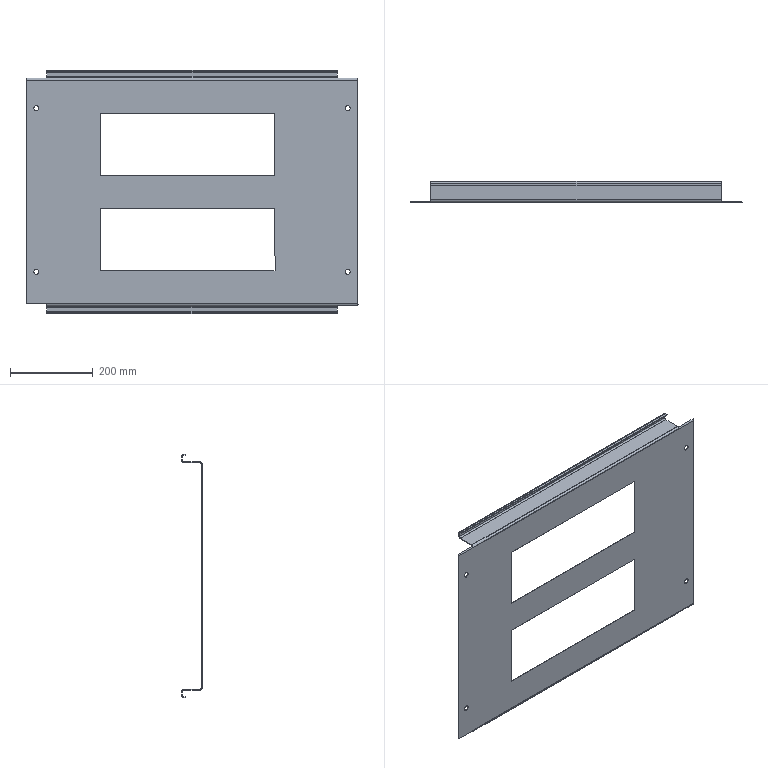Component | SolidWorks | LowerBaffle-2 | 1 solid | 71 faces | volume 816647 mm3 | plane 51 | cylinder 20 | commonest cylinder face diameters 12.5 x8 7 x6 11 x6